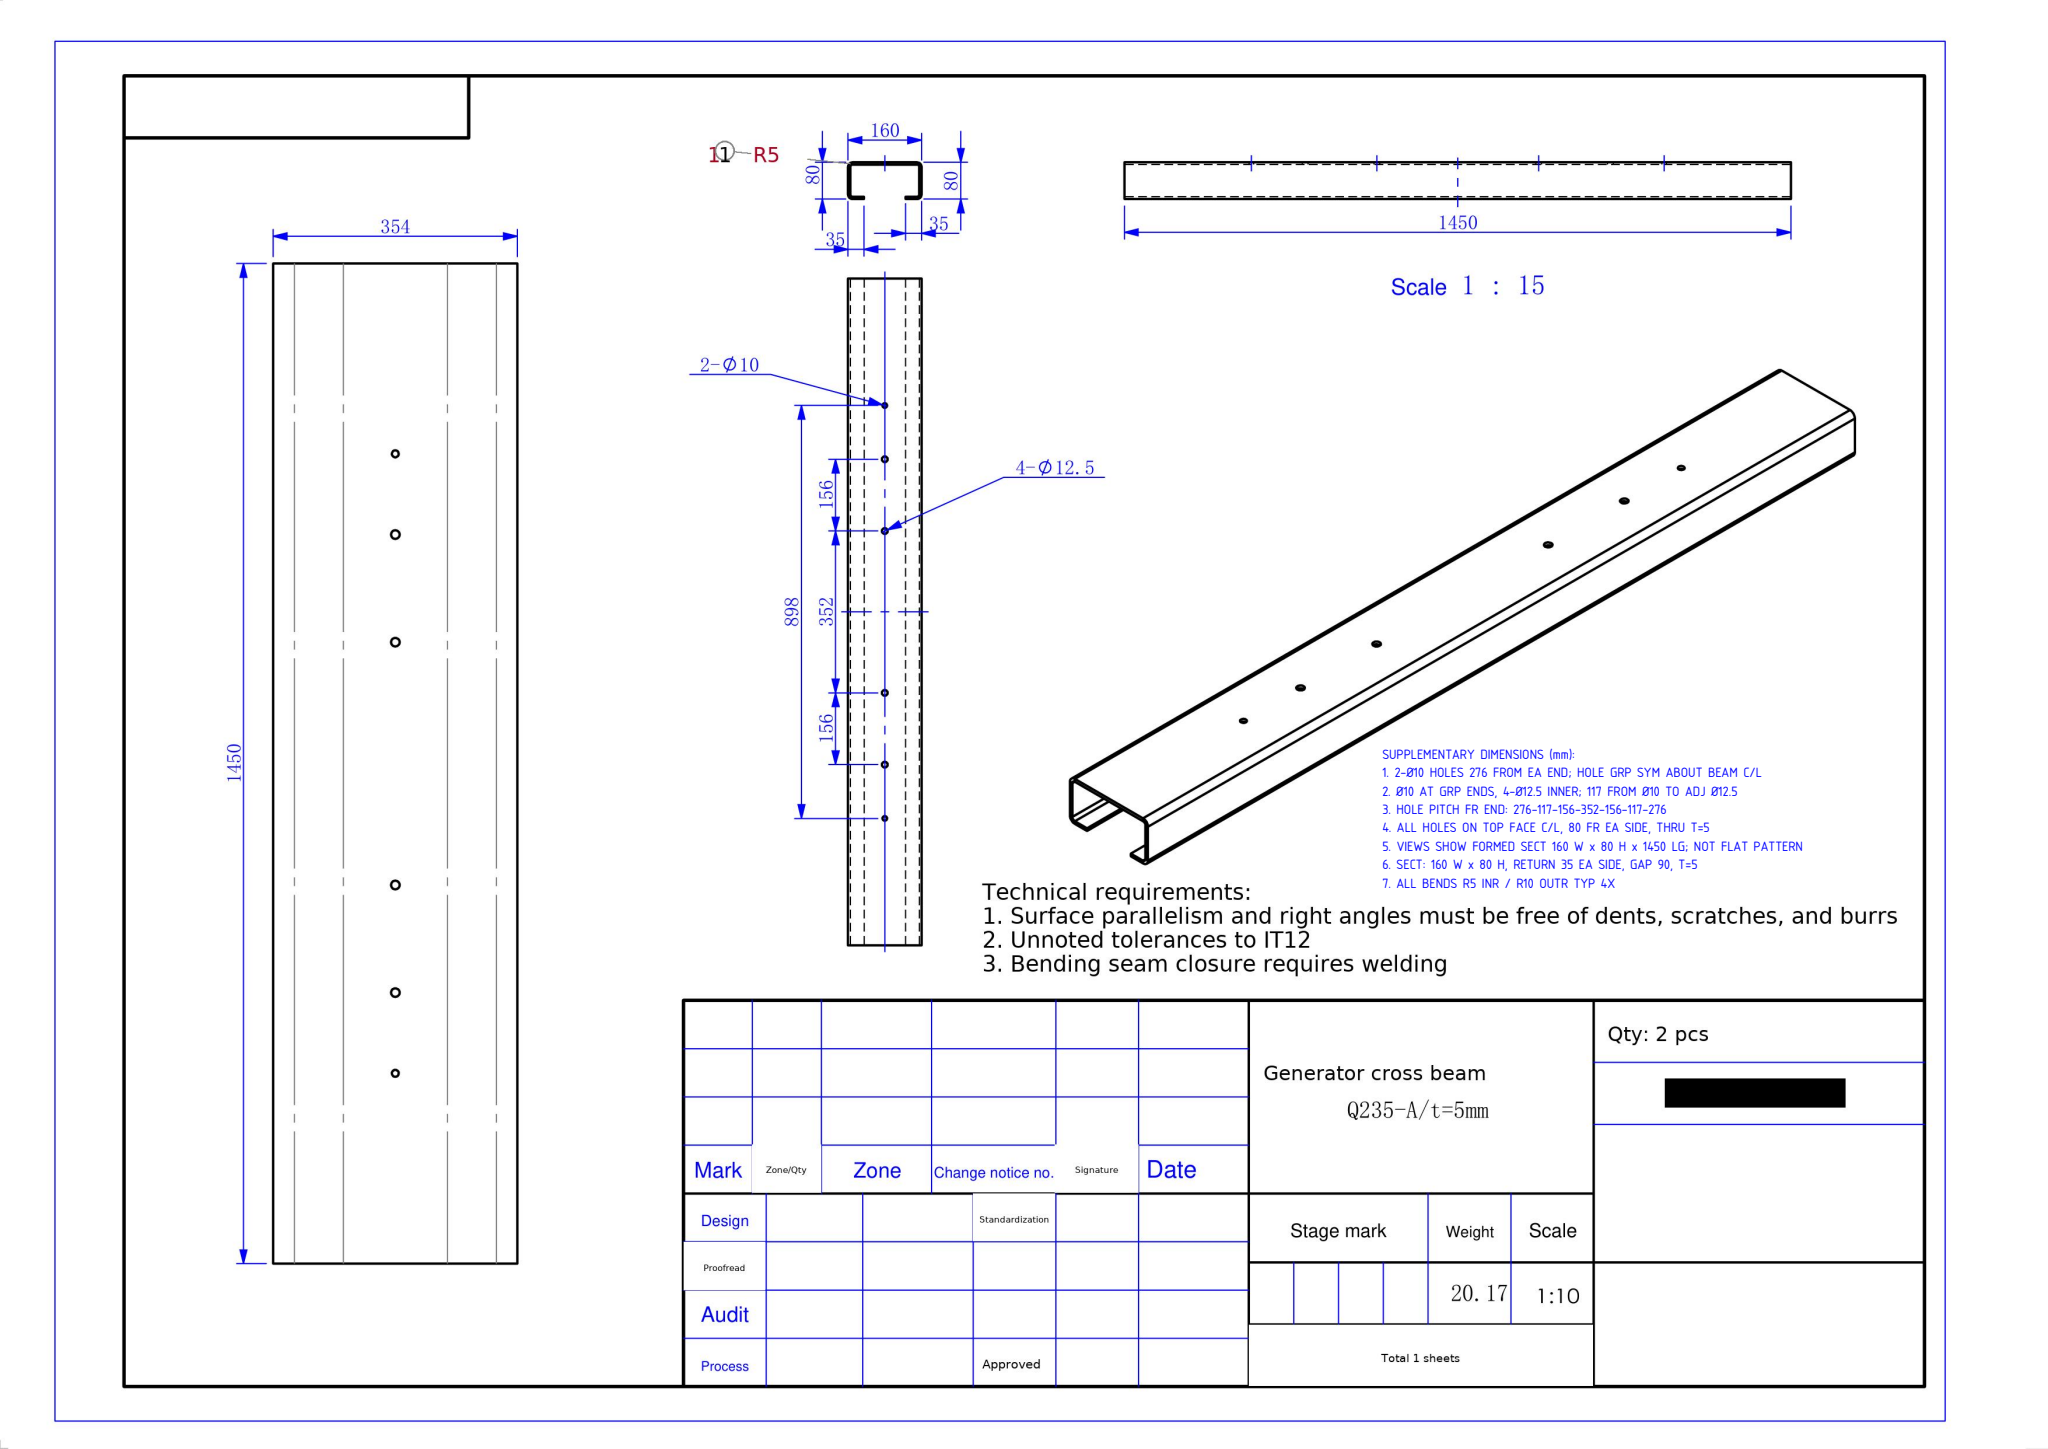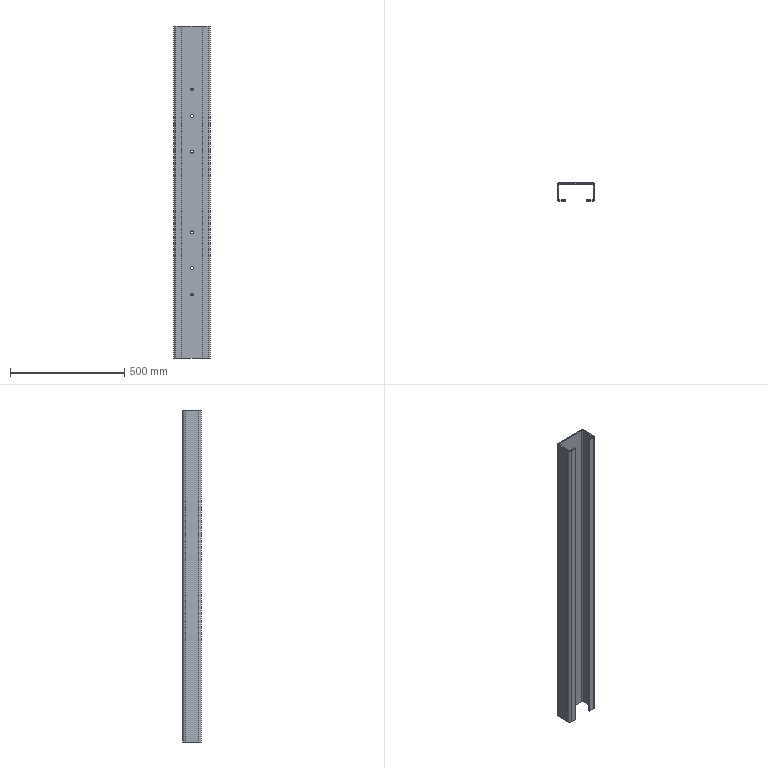Part | SolidWorks | mm | 1 solid | 50 faces | box 160 x 80 x 1450 mm | volume 2585908 mm3 | plane 30 | cylinder 20 | commonest cylinder face diameters 10 x8 12.5 x8 20 x4